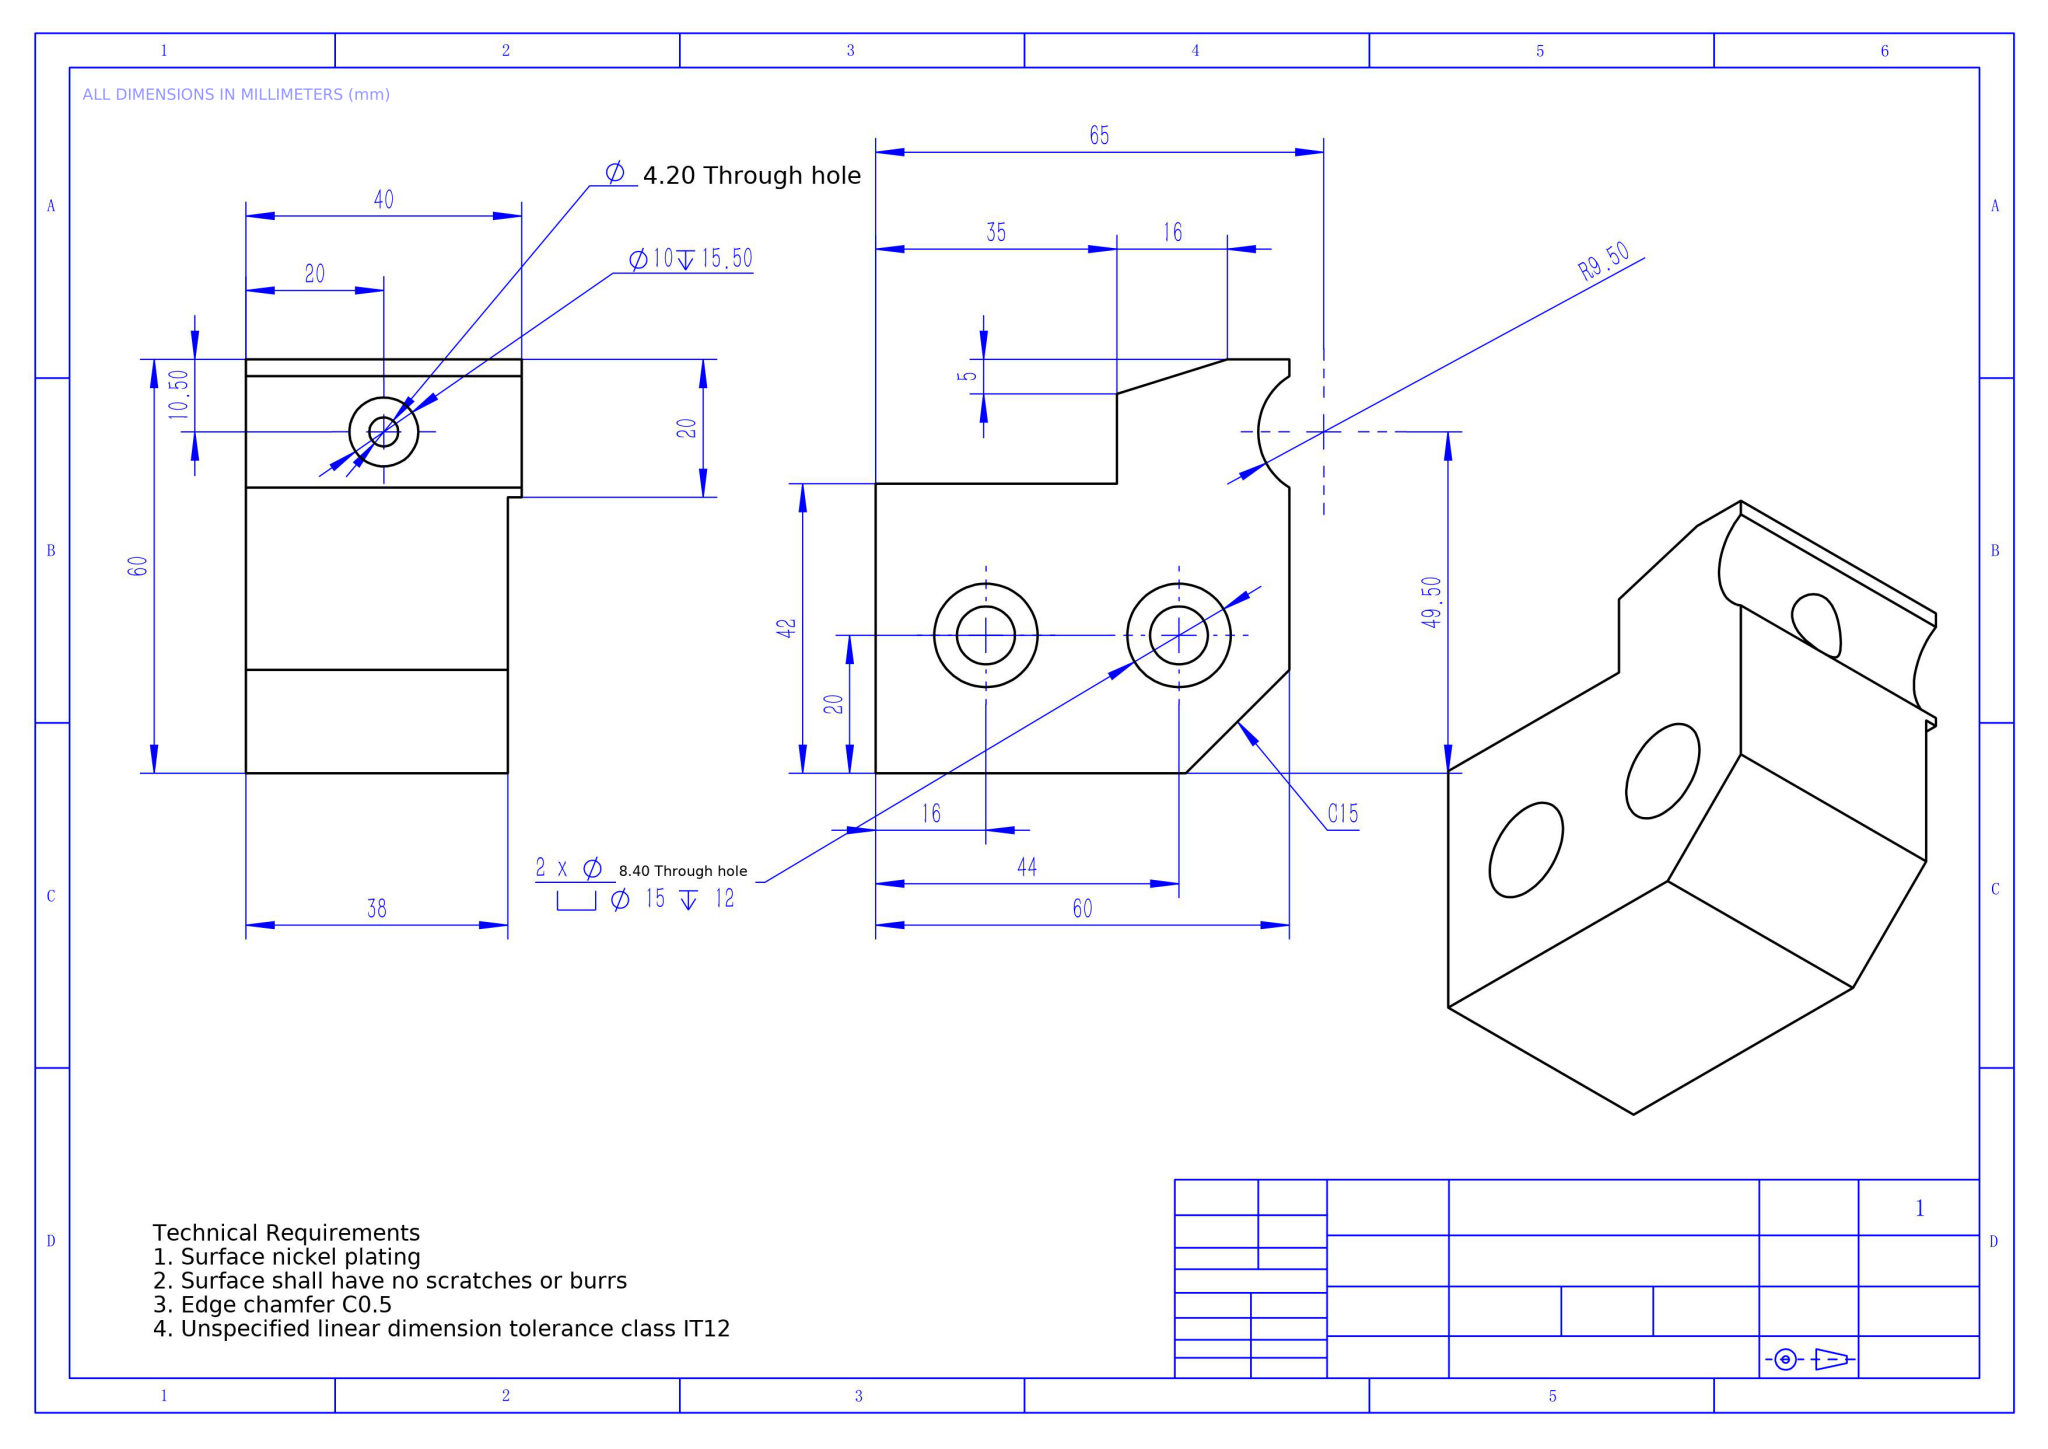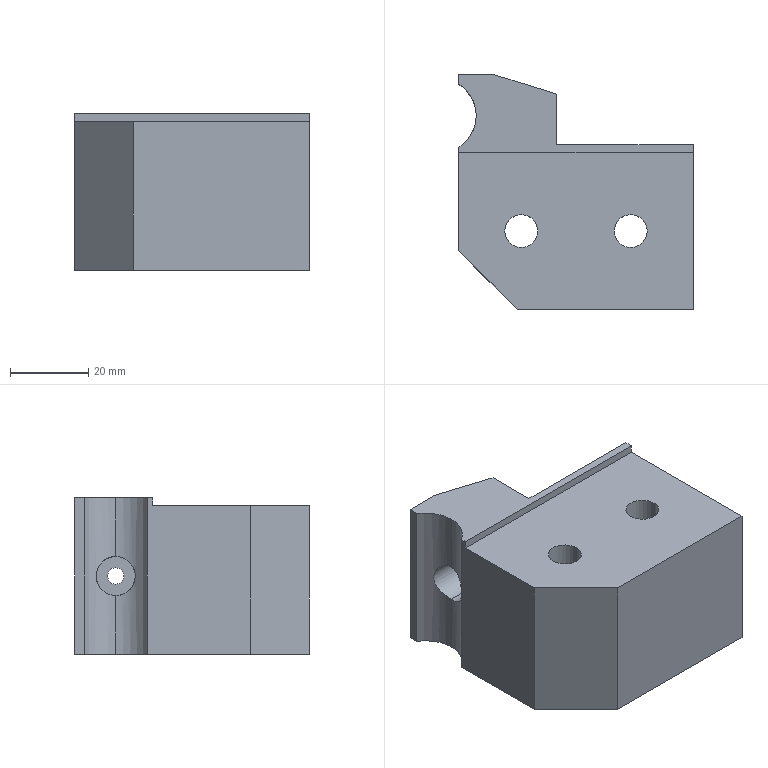Part | NX | mm | 1 solid | 30 faces | box 60 x 60 x 40 mm | volume 97635 mm3 | plane 16 | cylinder 14 | commonest cylinder face diameters 15 x4 8.4 x4 10 x2 19 x2 4.2 x2
STEP:
#1=COLOUR_RGB('',0.698,0.698,0.698);
#2=FILL_AREA_STYLE_COLOUR('',#1);
#3=FILL_AREA_STYLE('',(#2));
#4=SURFACE_STYLE_FILL_AREA(#3);
#5=SURFACE_SIDE_STYLE('',(#4));
#6=SURFACE_STYLE_USAGE(.BOTH.,#5);
#7=PRESENTATION_STYLE_ASSIGNMENT((#6));
#8=CARTESIAN_POINT('',(20.,49.5,15.));
#9=VERTEX_POINT('',#8);
#10=CARTESIAN_POINT('',(20.,49.5,25.));
#11=VERTEX_POINT('',#10);
#12=CARTESIAN_POINT('',(20.,49.5,20.));
#13=DIRECTION('',(-1.,0.,0.));
#14=DIRECTION('',(0.,0.,1.));
#15=AXIS2_PLACEMENT_3D('',#12,#13,#14);
#16=CIRCLE('',#15,5.);
#17=EDGE_CURVE('',#9,#11,#16,.T.);
#18=ORIENTED_EDGE('',*,*,#17,.F.);
#19=CARTESIAN_POINT('',(4.5,49.5,15.));
#20=VERTEX_POINT('',#19);
#21=CARTESIAN_POINT('',(20.,49.5,15.));
#22=DIRECTION('',(-1.,0.,0.));
#23=VECTOR('',#22,1000.);
#24=LINE('',#21,#23);
#25=EDGE_CURVE('',#9,#20,#24,.T.);
#26=ORIENTED_EDGE('',*,*,#25,.T.);
#27=CARTESIAN_POINT('',(4.5,49.5,25.));
#28=VERTEX_POINT('',#27);
#29=CARTESIAN_POINT('',(4.5,49.5,25.));
#30=CARTESIAN_POINT('',(4.5,49.163,25.));
#31=CARTESIAN_POINT('',(4.482,48.832,24.966));
#32=CARTESIAN_POINT('',(4.414,48.184,24.835));
#33=CARTESIAN_POINT('',(4.363,47.863,24.736));
#34=CARTESIAN_POINT('',(4.237,47.259,24.482));
#35=CARTESIAN_POINT('',(4.162,46.974,24.327));
#36=CARTESIAN_POINT('',(3.996,46.435,23.964));
#37=CARTESIAN_POINT('',(3.906,46.186,23.757));
#38=CARTESIAN_POINT('',(3.725,45.734,23.304));
#39=CARTESIAN_POINT('',(3.632,45.528,23.054));
#40=CARTESIAN_POINT('',(3.457,45.168,22.518));
#41=CARTESIAN_POINT('',(3.376,45.015,22.234));
#42=CARTESIAN_POINT('',(3.237,44.764,21.636));
#43=CARTESIAN_POINT('',(3.178,44.665,21.316));
#44=CARTESIAN_POINT('',(3.099,44.534,20.668));
#45=CARTESIAN_POINT('',(3.078,44.5,20.339));
#46=CARTESIAN_POINT('',(3.078,44.5,19.839));
#47=CARTESIAN_POINT('',(3.083,44.508,19.67));
#48=CARTESIAN_POINT('',(3.103,44.541,19.337));
#49=CARTESIAN_POINT('',(3.118,44.566,19.172));
#50=CARTESIAN_POINT('',(3.158,44.632,18.848));
#51=CARTESIAN_POINT('',(3.182,44.672,18.689));
#52=CARTESIAN_POINT('',(3.238,44.769,18.373));
#53=CARTESIAN_POINT('',(3.271,44.826,18.217));
#54=CARTESIAN_POINT('',(3.376,45.016,17.764));
#55=CARTESIAN_POINT('',(3.458,45.17,17.479));
#56=CARTESIAN_POINT('',(3.633,45.53,16.943));
#57=CARTESIAN_POINT('',(3.726,45.737,16.692));
#58=CARTESIAN_POINT('',(3.908,46.19,16.239));
#59=CARTESIAN_POINT('',(3.997,46.438,16.034));
#60=CARTESIAN_POINT('',(4.164,46.979,15.67));
#61=CARTESIAN_POINT('',(4.238,47.264,15.516));
#62=CARTESIAN_POINT('',(4.332,47.714,15.327));
#63=CARTESIAN_POINT('',(4.36,47.868,15.271));
#64=CARTESIAN_POINT('',(4.41,48.184,15.173));
#65=CARTESIAN_POINT('',(4.431,48.347,15.132));
#66=CARTESIAN_POINT('',(4.483,48.837,15.033));
#67=CARTESIAN_POINT('',(4.5,49.167,15.));
#68=CARTESIAN_POINT('',(4.5,49.5,15.));
#69=B_SPLINE_CURVE_WITH_KNOTS('',3,(#29,#30,#31,#32,#33,#34,#35,#36,#37,#38,#39,#40,#41,#42,#43,#44,#45,#46,#47,#48,#49,#50,#51,#52,#53,#54,#55,#56,#57,#58,#59,#60,#61,#62,#63,#64,#65,#66,#67,#68),.UNSPECIFIED.,.F.,.F.,(4,2,2,2,2,2,2,2,2,2,2,2,2,2,2,2,2,2,2,4),(0.,0.0009961,0.001992,0.002988,0.003985,0.004981,0.005977,0.006973,0.007969,0.008467,0.008965,0.009463,0.009961,0.01096,0.01195,0.01295,0.01395,0.01444,0.01494,0.01594),.UNSPECIFIED.);
#70=EDGE_CURVE('',#28,#20,#69,.T.);
#71=ORIENTED_EDGE('',*,*,#70,.F.);
#72=CARTESIAN_POINT('',(20.,49.5,25.));
#73=DIRECTION('',(-1.,0.,0.));
#74=VECTOR('',#73,1000.);
#75=LINE('',#72,#74);
#76=EDGE_CURVE('',#11,#28,#75,.T.);
#77=ORIENTED_EDGE('',*,*,#76,.F.);
#78=EDGE_LOOP('',(#18,#26,#71,#77));
#79=FACE_OUTER_BOUND('',#78,.T.);
#80=CARTESIAN_POINT('',(20.,49.5,20.));
#81=DIRECTION('',(-1.,0.,0.));
#82=DIRECTION('',(0.,0.,1.));
#83=AXIS2_PLACEMENT_3D('',#80,#81,#82);
#84=CYLINDRICAL_SURFACE('',#83,5.);
#85=ADVANCED_FACE('',(#79),#84,.F.);
#86=CARTESIAN_POINT('',(51.5,20.,12.));
#87=VERTEX_POINT('',#86);
#88=CARTESIAN_POINT('',(36.5,20.,12.));
#89=VERTEX_POINT('',#88);
#90=CARTESIAN_POINT('',(44.,20.,12.));
#91=DIRECTION('',(0.,0.,-1.));
#92=DIRECTION('',(-1.,0.,0.));
#93=AXIS2_PLACEMENT_3D('',#90,#91,#92);
#94=CIRCLE('',#93,7.5);
#95=EDGE_CURVE('',#87,#89,#94,.T.);
#96=ORIENTED_EDGE('',*,*,#95,.F.);
#97=CARTESIAN_POINT('',(51.5,20.,0.));
#98=VERTEX_POINT('',#97);
#99=CARTESIAN_POINT('',(51.5,20.,0.));
#100=DIRECTION('',(0.,0.,-1.));
#101=VECTOR('',#100,1000.);
#102=LINE('',#99,#101);
#103=EDGE_CURVE('',#87,#98,#102,.T.);
#104=ORIENTED_EDGE('',*,*,#103,.T.);
#105=CARTESIAN_POINT('',(36.5,20.,0.));
#106=VERTEX_POINT('',#105);
#107=CARTESIAN_POINT('',(44.,20.,0.));
#108=DIRECTION('',(0.,0.,-1.));
#109=DIRECTION('',(-1.,0.,0.));
#110=AXIS2_PLACEMENT_3D('',#107,#108,#109);
#111=CIRCLE('',#110,7.5);
#112=EDGE_CURVE('',#98,#106,#111,.T.);
#113=ORIENTED_EDGE('',*,*,#112,.T.);
#114=CARTESIAN_POINT('',(36.5,20.,0.));
#115=DIRECTION('',(0.,0.,-1.));
#116=VECTOR('',#115,1000.);
#117=LINE('',#114,#116);
#118=EDGE_CURVE('',#89,#106,#117,.T.);
#119=ORIENTED_EDGE('',*,*,#118,.F.);
#120=EDGE_LOOP('',(#96,#104,#113,#119));
#121=FACE_OUTER_BOUND('',#120,.T.);
#122=CARTESIAN_POINT('',(44.,20.,0.));
#123=DIRECTION('',(0.,0.,-1.));
#124=DIRECTION('',(-1.,0.,0.));
#125=AXIS2_PLACEMENT_3D('',#122,#123,#124);
#126=CYLINDRICAL_SURFACE('',#125,7.5);
#127=ADVANCED_FACE('',(#121),#126,.F.);
#128=CARTESIAN_POINT('',(39.8,20.,38.));
#129=VERTEX_POINT('',#128);
#130=CARTESIAN_POINT('',(48.2,20.,38.));
#131=VERTEX_POINT('',#130);
#132=CARTESIAN_POINT('',(44.,20.,38.));
#133=DIRECTION('',(0.,0.,1.));
#134=DIRECTION('',(1.,0.,0.));
#135=AXIS2_PLACEMENT_3D('',#132,#133,#134);
#136=CIRCLE('',#135,4.2);
#137=EDGE_CURVE('',#129,#131,#136,.T.);
#138=ORIENTED_EDGE('',*,*,#137,.T.);
#139=CARTESIAN_POINT('',(48.2,20.,12.));
#140=VERTEX_POINT('',#139);
#141=CARTESIAN_POINT('',(48.2,20.,0.));
#142=DIRECTION('',(0.,0.,-1.));
#143=VECTOR('',#142,1000.);
#144=LINE('',#141,#143);
#145=EDGE_CURVE('',#131,#140,#144,.T.);
#146=ORIENTED_EDGE('',*,*,#145,.T.);
#147=CARTESIAN_POINT('',(39.8,20.,12.));
#148=VERTEX_POINT('',#147);
#149=CARTESIAN_POINT('',(44.,20.,12.));
#150=DIRECTION('',(0.,0.,-1.));
#151=DIRECTION('',(-1.,0.,0.));
#152=AXIS2_PLACEMENT_3D('',#149,#150,#151);
#153=CIRCLE('',#152,4.2);
#154=EDGE_CURVE('',#140,#148,#153,.T.);
#155=ORIENTED_EDGE('',*,*,#154,.T.);
#156=CARTESIAN_POINT('',(39.8,20.,0.));
#157=DIRECTION('',(0.,0.,-1.));
#158=VECTOR('',#157,1000.);
#159=LINE('',#156,#158);
#160=EDGE_CURVE('',#129,#148,#159,.T.);
#161=ORIENTED_EDGE('',*,*,#160,.F.);
#162=EDGE_LOOP('',(#138,#146,#155,#161));
#163=FACE_OUTER_BOUND('',#162,.T.);
#164=CARTESIAN_POINT('',(44.,20.,0.));
#165=DIRECTION('',(0.,0.,-1.));
#166=DIRECTION('',(-1.,0.,0.));
#167=AXIS2_PLACEMENT_3D('',#164,#165,#166);
#168=CYLINDRICAL_SURFACE('',#167,4.2);
#169=ADVANCED_FACE('',(#163),#168,.F.);
#170=CARTESIAN_POINT('',(23.5,20.,12.));
#171=VERTEX_POINT('',#170);
#172=CARTESIAN_POINT('',(8.5,20.,12.));
#173=VERTEX_POINT('',#172);
#174=CARTESIAN_POINT('',(16.,20.,12.));
#175=DIRECTION('',(0.,0.,-1.));
#176=DIRECTION('',(-1.,0.,0.));
#177=AXIS2_PLACEMENT_3D('',#174,#175,#176);
#178=CIRCLE('',#177,7.5);
#179=EDGE_CURVE('',#171,#173,#178,.T.);
#180=ORIENTED_EDGE('',*,*,#179,.F.);
#181=CARTESIAN_POINT('',(23.5,20.,0.));
#182=VERTEX_POINT('',#181);
#183=CARTESIAN_POINT('',(23.5,20.,0.));
#184=DIRECTION('',(0.,0.,-1.));
#185=VECTOR('',#184,1000.);
#186=LINE('',#183,#185);
#187=EDGE_CURVE('',#171,#182,#186,.T.);
#188=ORIENTED_EDGE('',*,*,#187,.T.);
#189=CARTESIAN_POINT('',(8.5,20.,0.));
#190=VERTEX_POINT('',#189);
#191=CARTESIAN_POINT('',(16.,20.,0.));
#192=DIRECTION('',(0.,0.,-1.));
#193=DIRECTION('',(-1.,0.,0.));
#194=AXIS2_PLACEMENT_3D('',#191,#192,#193);
#195=CIRCLE('',#194,7.5);
#196=EDGE_CURVE('',#182,#190,#195,.T.);
#197=ORIENTED_EDGE('',*,*,#196,.T.);
#198=CARTESIAN_POINT('',(8.5,20.,0.));
#199=DIRECTION('',(0.,0.,-1.));
#200=VECTOR('',#199,1000.);
#201=LINE('',#198,#200);
#202=EDGE_CURVE('',#173,#190,#201,.T.);
#203=ORIENTED_EDGE('',*,*,#202,.F.);
#204=EDGE_LOOP('',(#180,#188,#197,#203));
#205=FACE_OUTER_BOUND('',#204,.T.);
#206=CARTESIAN_POINT('',(16.,20.,0.));
#207=DIRECTION('',(0.,0.,-1.));
#208=DIRECTION('',(-1.,0.,0.));
#209=AXIS2_PLACEMENT_3D('',#206,#207,#208);
#210=CYLINDRICAL_SURFACE('',#209,7.5);
#211=ADVANCED_FACE('',(#205),#210,.F.);
#212=CARTESIAN_POINT('',(11.8,20.,38.));
#213=VERTEX_POINT('',#212);
#214=CARTESIAN_POINT('',(20.2,20.,38.));
#215=VERTEX_POINT('',#214);
#216=CARTESIAN_POINT('',(16.,20.,38.));
#217=DIRECTION('',(0.,0.,1.));
#218=DIRECTION('',(1.,0.,0.));
#219=AXIS2_PLACEMENT_3D('',#216,#217,#218);
#220=CIRCLE('',#219,4.2);
#221=EDGE_CURVE('',#213,#215,#220,.T.);
#222=ORIENTED_EDGE('',*,*,#221,.T.);
#223=CARTESIAN_POINT('',(20.2,20.,12.));
#224=VERTEX_POINT('',#223);
#225=CARTESIAN_POINT('',(20.2,20.,0.));
#226=DIRECTION('',(0.,0.,-1.));
#227=VECTOR('',#226,1000.);
#228=LINE('',#225,#227);
#229=EDGE_CURVE('',#215,#224,#228,.T.);
#230=ORIENTED_EDGE('',*,*,#229,.T.);
#231=CARTESIAN_POINT('',(11.8,20.,12.));
#232=VERTEX_POINT('',#231);
#233=CARTESIAN_POINT('',(16.,20.,12.));
#234=DIRECTION('',(0.,0.,-1.));
#235=DIRECTION('',(-1.,0.,0.));
#236=AXIS2_PLACEMENT_3D('',#233,#234,#235);
#237=CIRCLE('',#236,4.2);
#238=EDGE_CURVE('',#224,#232,#237,.T.);
#239=ORIENTED_EDGE('',*,*,#238,.T.);
#240=CARTESIAN_POINT('',(11.8,20.,0.));
#241=DIRECTION('',(0.,0.,-1.));
#242=VECTOR('',#241,1000.);
#243=LINE('',#240,#242);
#244=EDGE_CURVE('',#213,#232,#243,.T.);
#245=ORIENTED_EDGE('',*,*,#244,.F.);
#246=EDGE_LOOP('',(#222,#230,#239,#245));
#247=FACE_OUTER_BOUND('',#246,.T.);
#248=CARTESIAN_POINT('',(16.,20.,0.));
#249=DIRECTION('',(0.,0.,-1.));
#250=DIRECTION('',(-1.,0.,0.));
#251=AXIS2_PLACEMENT_3D('',#248,#249,#250);
#252=CYLINDRICAL_SURFACE('',#251,4.2);
#253=ADVANCED_FACE('',(#247),#252,.F.);
#254=CARTESIAN_POINT('',(0.,57.578,0.));
#255=VERTEX_POINT('',#254);
#256=CARTESIAN_POINT('',(4.5,49.5,0.));
#257=VERTEX_POINT('',#256);
#258=CARTESIAN_POINT('',(-5.,49.5,0.));
#259=DIRECTION('',(0.,0.,-1.));
#260=DIRECTION('',(-1.,0.,0.));
#261=AXIS2_PLACEMENT_3D('',#258,#259,#260);
#262=CIRCLE('',#261,9.5);
#263=EDGE_CURVE('',#255,#257,#262,.T.);
#264=ORIENTED_EDGE('',*,*,#263,.T.);
#265=CARTESIAN_POINT('',(4.5,49.5,0.));
#266=DIRECTION('',(0.,0.,1.));
#267=VECTOR('',#266,1000.);
#268=LINE('',#265,#267);
#269=EDGE_CURVE('',#257,#20,#268,.T.);
#270=ORIENTED_EDGE('',*,*,#269,.T.);
#271=CARTESIAN_POINT('',(4.5,49.5,15.));
#272=CARTESIAN_POINT('',(4.5,49.832,15.));
#273=CARTESIAN_POINT('',(4.482,50.17,15.034));
#274=CARTESIAN_POINT('',(4.414,50.819,15.166));
#275=CARTESIAN_POINT('',(4.363,51.135,15.263));
#276=CARTESIAN_POINT('',(4.237,51.743,15.519));
#277=CARTESIAN_POINT('',(4.162,52.028,15.674));
#278=CARTESIAN_POINT('',(3.997,52.563,16.035));
#279=CARTESIAN_POINT('',(3.906,52.815,16.243));
#280=CARTESIAN_POINT('',(3.725,53.267,16.697));
#281=CARTESIAN_POINT('',(3.633,53.47,16.943));
#282=CARTESIAN_POINT('',(3.458,53.83,17.48));
#283=CARTESIAN_POINT('',(3.376,53.985,17.767));
#284=CARTESIAN_POINT('',(3.237,54.236,18.364));
#285=CARTESIAN_POINT('',(3.179,54.333,18.676));
#286=CARTESIAN_POINT('',(3.099,54.466,19.331));
#287=CARTESIAN_POINT('',(3.078,54.5,19.662));
#288=CARTESIAN_POINT('',(3.078,54.5,20.159));
#289=CARTESIAN_POINT('',(3.083,54.492,20.325));
#290=CARTESIAN_POINT('',(3.103,54.459,20.658));
#291=CARTESIAN_POINT('',(3.118,54.434,20.824));
#292=CARTESIAN_POINT('',(3.177,54.336,21.312));
#293=CARTESIAN_POINT('',(3.234,54.24,21.626));
#294=CARTESIAN_POINT('',(3.375,53.986,22.232));
#295=CARTESIAN_POINT('',(3.457,53.832,22.518));
#296=CARTESIAN_POINT('',(3.632,53.473,23.052));
#297=CARTESIAN_POINT('',(3.725,53.267,23.304));
#298=CARTESIAN_POINT('',(3.907,52.813,23.759));
#299=CARTESIAN_POINT('',(3.996,52.566,23.962));
#300=CARTESIAN_POINT('',(4.161,52.031,24.324));
#301=CARTESIAN_POINT('',(4.237,51.74,24.482));
#302=CARTESIAN_POINT('',(4.362,51.14,24.735));
#303=CARTESIAN_POINT('',(4.413,50.827,24.832));
#304=CARTESIAN_POINT('',(4.482,50.174,24.966));
#305=CARTESIAN_POINT('',(4.5,49.837,25.));
#306=CARTESIAN_POINT('',(4.5,49.5,25.));
#307=B_SPLINE_CURVE_WITH_KNOTS('',3,(#271,#272,#273,#274,#275,#276,#277,#278,#279,#280,#281,#282,#283,#284,#285,#286,#287,#288,#289,#290,#291,#292,#293,#294,#295,#296,#297,#298,#299,#300,#301,#302,#303,#304,#305,#306),.UNSPECIFIED.,.F.,.F.,(4,2,2,2,2,2,2,2,2,2,2,2,2,2,2,2,2,4),(0.01594,0.01693,0.01793,0.01892,0.01991,0.02091,0.0219,0.0229,0.02389,0.02439,0.02488,0.02588,0.02687,0.02787,0.02886,0.02986,0.03085,0.03184),.UNSPECIFIED.);
#308=EDGE_CURVE('',#20,#28,#307,.T.);
#309=ORIENTED_EDGE('',*,*,#308,.T.);
#310=CARTESIAN_POINT('',(4.5,49.5,40.));
#311=VERTEX_POINT('',#310);
#312=CARTESIAN_POINT('',(4.5,49.5,0.));
#313=DIRECTION('',(0.,0.,1.));
#314=VECTOR('',#313,1000.);
#315=LINE('',#312,#314);
#316=EDGE_CURVE('',#28,#311,#315,.T.);
#317=ORIENTED_EDGE('',*,*,#316,.T.);
#318=CARTESIAN_POINT('',(-0.,57.578,40.));
#319=VERTEX_POINT('',#318);
#320=CARTESIAN_POINT('',(-5.,49.5,40.));
#321=DIRECTION('',(0.,0.,1.));
#322=DIRECTION('',(1.,0.,0.));
#323=AXIS2_PLACEMENT_3D('',#320,#321,#322);
#324=CIRCLE('',#323,9.5);
#325=EDGE_CURVE('',#311,#319,#324,.T.);
#326=ORIENTED_EDGE('',*,*,#325,.T.);
#327=CARTESIAN_POINT('',(0.,57.578,0.));
#328=DIRECTION('',(0.,0.,1.));
#329=VECTOR('',#328,1000.);
#330=LINE('',#327,#329);
#331=EDGE_CURVE('',#255,#319,#330,.T.);
#332=ORIENTED_EDGE('',*,*,#331,.F.);
#333=EDGE_LOOP('',(#264,#270,#309,#317,#326,#332));
#334=FACE_OUTER_BOUND('',#333,.T.);
#335=CARTESIAN_POINT('',(-5.,49.5,0.));
#336=DIRECTION('',(0.,0.,1.));
#337=DIRECTION('',(1.,0.,0.));
#338=AXIS2_PLACEMENT_3D('',#335,#336,#337);
#339=CYLINDRICAL_SURFACE('',#338,9.5);
#340=ADVANCED_FACE('',(#334),#339,.F.);
#341=CARTESIAN_POINT('',(20.,49.5,22.1));
#342=VERTEX_POINT('',#341);
#343=CARTESIAN_POINT('',(20.,49.5,17.9));
#344=VERTEX_POINT('',#343);
#345=CARTESIAN_POINT('',(20.,49.5,20.));
#346=DIRECTION('',(1.,0.,0.));
#347=DIRECTION('',(0.,0.,1.));
#348=AXIS2_PLACEMENT_3D('',#345,#346,#347);
#349=CIRCLE('',#348,2.1);
#350=EDGE_CURVE('',#342,#344,#349,.T.);
#351=ORIENTED_EDGE('',*,*,#350,.F.);
#352=CARTESIAN_POINT('',(25.,49.5,22.1));
#353=VERTEX_POINT('',#352);
#354=CARTESIAN_POINT('',(25.,49.5,22.1));
#355=DIRECTION('',(1.,0.,0.));
#356=VECTOR('',#355,1000.);
#357=LINE('',#354,#356);
#358=EDGE_CURVE('',#342,#353,#357,.T.);
#359=ORIENTED_EDGE('',*,*,#358,.T.);
#360=CARTESIAN_POINT('',(25.,49.5,17.9));
#361=VERTEX_POINT('',#360);
#362=CARTESIAN_POINT('',(25.,49.5,20.));
#363=DIRECTION('',(1.,0.,0.));
#364=DIRECTION('',(0.,0.,-1.));
#365=AXIS2_PLACEMENT_3D('',#362,#363,#364);
#366=CIRCLE('',#365,2.1);
#367=EDGE_CURVE('',#353,#361,#366,.T.);
#368=ORIENTED_EDGE('',*,*,#367,.T.);
#369=CARTESIAN_POINT('',(25.,49.5,17.9));
#370=DIRECTION('',(1.,0.,0.));
#371=VECTOR('',#370,1000.);
#372=LINE('',#369,#371);
#373=EDGE_CURVE('',#344,#361,#372,.T.);
#374=ORIENTED_EDGE('',*,*,#373,.F.);
#375=EDGE_LOOP('',(#351,#359,#368,#374));
#376=FACE_OUTER_BOUND('',#375,.T.);
#377=CARTESIAN_POINT('',(25.,49.5,20.));
#378=DIRECTION('',(1.,0.,0.));
#379=DIRECTION('',(0.,0.,-1.));
#380=AXIS2_PLACEMENT_3D('',#377,#378,#379);
#381=CYLINDRICAL_SURFACE('',#380,2.1);
#382=ADVANCED_FACE('',(#376),#381,.F.);
#383=ORIENTED_EDGE('',*,*,#358,.F.);
#384=CARTESIAN_POINT('',(20.,49.5,20.));
#385=DIRECTION('',(1.,0.,0.));
#386=DIRECTION('',(0.,0.,1.));
#387=AXIS2_PLACEMENT_3D('',#384,#385,#386);
#388=CIRCLE('',#387,2.1);
#389=EDGE_CURVE('',#344,#342,#388,.T.);
#390=ORIENTED_EDGE('',*,*,#389,.F.);
#391=ORIENTED_EDGE('',*,*,#373,.T.);
#392=CARTESIAN_POINT('',(25.,49.5,20.));
#393=DIRECTION('',(1.,0.,0.));
#394=DIRECTION('',(0.,0.,-1.));
#395=AXIS2_PLACEMENT_3D('',#392,#393,#394);
#396=CIRCLE('',#395,2.1);
#397=EDGE_CURVE('',#361,#353,#396,.T.);
#398=ORIENTED_EDGE('',*,*,#397,.T.);
#399=EDGE_LOOP('',(#383,#390,#391,#398));
#400=FACE_OUTER_BOUND('',#399,.T.);
#401=CARTESIAN_POINT('',(25.,49.5,20.));
#402=DIRECTION('',(1.,0.,0.));
#403=DIRECTION('',(0.,0.,-1.));
#404=AXIS2_PLACEMENT_3D('',#401,#402,#403);
#405=CYLINDRICAL_SURFACE('',#404,2.1);
#406=ADVANCED_FACE('',(#400),#405,.F.);
#407=CARTESIAN_POINT('',(15.,-0.,38.));
#408=VERTEX_POINT('',#407);
#409=CARTESIAN_POINT('',(60.,0.,38.));
#410=VERTEX_POINT('',#409);
#411=CARTESIAN_POINT('',(60.,0.,38.));
#412=DIRECTION('',(1.,0.,0.));
#413=VECTOR('',#412,1000.);
#414=LINE('',#411,#413);
#415=EDGE_CURVE('',#408,#410,#414,.T.);
#416=ORIENTED_EDGE('',*,*,#415,.F.);
#417=CARTESIAN_POINT('',(15.,0.,0.));
#418=VERTEX_POINT('',#417);
#419=CARTESIAN_POINT('',(15.,0.,40.));
#420=DIRECTION('',(0.,0.,-1.));
#421=VECTOR('',#420,1000.);
#422=LINE('',#419,#421);
#423=EDGE_CURVE('',#408,#418,#422,.T.);
#424=ORIENTED_EDGE('',*,*,#423,.T.);
#425=CARTESIAN_POINT('',(60.,0.,0.));
#426=VERTEX_POINT('',#425);
#427=CARTESIAN_POINT('',(0.,0.,0.));
#428=DIRECTION('',(1.,0.,0.));
#429=VECTOR('',#428,1000.);
#430=LINE('',#427,#429);
#431=EDGE_CURVE('',#418,#426,#430,.T.);
#432=ORIENTED_EDGE('',*,*,#431,.T.);
#433=CARTESIAN_POINT('',(60.,0.,40.));
#434=DIRECTION('',(0.,0.,-1.));
#435=VECTOR('',#434,1000.);
#436=LINE('',#433,#435);
#437=EDGE_CURVE('',#410,#426,#436,.T.);
#438=ORIENTED_EDGE('',*,*,#437,.F.);
#439=EDGE_LOOP('',(#416,#424,#432,#438));
#440=FACE_OUTER_BOUND('',#439,.T.);
#441=CARTESIAN_POINT('',(0.,0.,40.));
#442=DIRECTION('',(0.,1.,0.));
#443=DIRECTION('',(0.,0.,1.));
#444=AXIS2_PLACEMENT_3D('',#441,#442,#443);
#445=PLANE('',#444);
#446=ADVANCED_FACE('',(#440),#445,.F.);
#447=ORIENTED_EDGE('',*,*,#423,.F.);
#448=CARTESIAN_POINT('',(0.,15.,38.));
#449=VERTEX_POINT('',#448);
#450=CARTESIAN_POINT('',(15.,0.,38.));
#451=DIRECTION('',(-0.7071,0.7071,0.));
#452=VECTOR('',#451,1000.);
#453=LINE('',#450,#452);
#454=EDGE_CURVE('',#408,#449,#453,.T.);
#455=ORIENTED_EDGE('',*,*,#454,.T.);
#456=CARTESIAN_POINT('',(0.,15.,0.));
#457=VERTEX_POINT('',#456);
#458=CARTESIAN_POINT('',(0.,15.,40.));
#459=DIRECTION('',(0.,0.,1.));
#460=VECTOR('',#459,1000.);
#461=LINE('',#458,#460);
#462=EDGE_CURVE('',#457,#449,#461,.T.);
#463=ORIENTED_EDGE('',*,*,#462,.F.);
#464=CARTESIAN_POINT('',(7.5,7.5,0.));
#465=DIRECTION('',(-0.7071,0.7071,0.));
#466=VECTOR('',#465,1000.);
#467=LINE('',#464,#466);
#468=EDGE_CURVE('',#418,#457,#467,.T.);
#469=ORIENTED_EDGE('',*,*,#468,.F.);
#470=EDGE_LOOP('',(#447,#455,#463,#469));
#471=FACE_OUTER_BOUND('',#470,.T.);
#472=CARTESIAN_POINT('',(15.,0.,40.));
#473=DIRECTION('',(0.7071,0.7071,0.));
#474=DIRECTION('',(0.,0.,-1.));
#475=AXIS2_PLACEMENT_3D('',#472,#473,#474);
#476=PLANE('',#475);
#477=ADVANCED_FACE('',(#471),#476,.F.);
#478=CARTESIAN_POINT('',(0.,60.,0.));
#479=VERTEX_POINT('',#478);
#480=CARTESIAN_POINT('',(0.,0.,0.));
#481=DIRECTION('',(0.,-1.,0.));
#482=VECTOR('',#481,1000.);
#483=LINE('',#480,#482);
#484=EDGE_CURVE('',#479,#255,#483,.T.);
#485=ORIENTED_EDGE('',*,*,#484,.T.);
#486=ORIENTED_EDGE('',*,*,#331,.T.);
#487=CARTESIAN_POINT('',(0.,60.,40.));
#488=VERTEX_POINT('',#487);
#489=CARTESIAN_POINT('',(0.,0.,40.));
#490=DIRECTION('',(0.,-1.,0.));
#491=VECTOR('',#490,1000.);
#492=LINE('',#489,#491);
#493=EDGE_CURVE('',#488,#319,#492,.T.);
#494=ORIENTED_EDGE('',*,*,#493,.F.);
#495=CARTESIAN_POINT('',(0.,60.,40.));
#496=DIRECTION('',(0.,0.,-1.));
#497=VECTOR('',#496,1000.);
#498=LINE('',#495,#497);
#499=EDGE_CURVE('',#488,#479,#498,.T.);
#500=ORIENTED_EDGE('',*,*,#499,.T.);
#501=EDGE_LOOP('',(#485,#486,#494,#500));
#502=FACE_OUTER_BOUND('',#501,.T.);
#503=CARTESIAN_POINT('',(0.,0.,40.));
#504=DIRECTION('',(1.,0.,0.));
#505=DIRECTION('',(0.,0.,-1.));
#506=AXIS2_PLACEMENT_3D('',#503,#504,#505);
#507=PLANE('',#506);
#508=ADVANCED_FACE('',(#502),#507,.F.);
#509=CARTESIAN_POINT('',(0.,40.,38.));
#510=VERTEX_POINT('',#509);
#511=CARTESIAN_POINT('',(0.,0.,38.));
#512=DIRECTION('',(0.,-1.,0.));
#513=VECTOR('',#512,1000.);
#514=LINE('',#511,#513);
#515=EDGE_CURVE('',#510,#449,#514,.T.);
#516=ORIENTED_EDGE('',*,*,#515,.F.);
#517=CARTESIAN_POINT('',(0.,40.,40.));
#518=VERTEX_POINT('',#517);
#519=CARTESIAN_POINT('',(0.,40.,40.));
#520=DIRECTION('',(0.,0.,1.));
#521=VECTOR('',#520,1000.);
#522=LINE('',#519,#521);
#523=EDGE_CURVE('',#510,#518,#522,.T.);
#524=ORIENTED_EDGE('',*,*,#523,.T.);
#525=CARTESIAN_POINT('',(-0.,41.422,40.));
#526=VERTEX_POINT('',#525);
#527=CARTESIAN_POINT('',(0.,0.,40.));
#528=DIRECTION('',(0.,-1.,0.));
#529=VECTOR('',#528,1000.);
#530=LINE('',#527,#529);
#531=EDGE_CURVE('',#526,#518,#530,.T.);
#532=ORIENTED_EDGE('',*,*,#531,.F.);
#533=CARTESIAN_POINT('',(-0.,41.422,0.));
#534=VERTEX_POINT('',#533);
#535=CARTESIAN_POINT('',(0.,41.422,0.));
#536=DIRECTION('',(0.,0.,-1.));
#537=VECTOR('',#536,1000.);
#538=LINE('',#535,#537);
#539=EDGE_CURVE('',#526,#534,#538,.T.);
#540=ORIENTED_EDGE('',*,*,#539,.T.);
#541=CARTESIAN_POINT('',(0.,0.,0.));
#542=DIRECTION('',(0.,-1.,0.));
#543=VECTOR('',#542,1000.);
#544=LINE('',#541,#543);
#545=EDGE_CURVE('',#534,#457,#544,.T.);
#546=ORIENTED_EDGE('',*,*,#545,.T.);
#547=ORIENTED_EDGE('',*,*,#462,.T.);
#548=EDGE_LOOP('',(#516,#524,#532,#540,#546,#547));
#549=FACE_OUTER_BOUND('',#548,.T.);
#550=CARTESIAN_POINT('',(0.,0.,40.));
#551=DIRECTION('',(1.,0.,0.));
#552=DIRECTION('',(0.,0.,-1.));
#553=AXIS2_PLACEMENT_3D('',#550,#551,#552);
#554=PLANE('',#553);
#555=ADVANCED_FACE('',(#549),#554,.F.);
#556=CARTESIAN_POINT('',(60.,40.,40.));
#557=VERTEX_POINT('',#556);
#558=CARTESIAN_POINT('',(60.,42.,40.));
#559=VERTEX_POINT('',#558);
#560=CARTESIAN_POINT('',(60.,0.,40.));
#561=DIRECTION('',(0.,1.,0.));
#562=VECTOR('',#561,1000.);
#563=LINE('',#560,#562);
#564=EDGE_CURVE('',#557,#559,#563,.T.);
#565=ORIENTED_EDGE('',*,*,#564,.F.);
#566=CARTESIAN_POINT('',(60.,40.,38.));
#567=VERTEX_POINT('',#566);
#568=CARTESIAN_POINT('',(60.,40.,38.));
#569=DIRECTION('',(0.,0.,1.));
#570=VECTOR('',#569,1000.);
#571=LINE('',#568,#570);
#572=EDGE_CURVE('',#567,#557,#571,.T.);
#573=ORIENTED_EDGE('',*,*,#572,.F.);
#574=CARTESIAN_POINT('',(60.,0.,38.));
#575=DIRECTION('',(0.,1.,0.));
#576=VECTOR('',#575,1000.);
#577=LINE('',#574,#576);
#578=EDGE_CURVE('',#410,#567,#577,.T.);
#579=ORIENTED_EDGE('',*,*,#578,.F.);
#580=ORIENTED_EDGE('',*,*,#437,.T.);
#581=CARTESIAN_POINT('',(60.,42.,0.));
#582=VERTEX_POINT('',#581);
#583=CARTESIAN_POINT('',(60.,0.,0.));
#584=DIRECTION('',(0.,1.,0.));
#585=VECTOR('',#584,1000.);
#586=LINE('',#583,#585);
#587=EDGE_CURVE('',#426,#582,#586,.T.);
#588=ORIENTED_EDGE('',*,*,#587,.T.);
#589=CARTESIAN_POINT('',(60.,42.,0.));
#590=DIRECTION('',(0.,0.,1.));
#591=VECTOR('',#590,1000.);
#592=LINE('',#589,#591);
#593=EDGE_CURVE('',#582,#559,#592,.T.);
#594=ORIENTED_EDGE('',*,*,#593,.T.);
#595=EDGE_LOOP('',(#565,#573,#579,#580,#588,#594));
#596=FACE_OUTER_BOUND('',#595,.T.);
#597=CARTESIAN_POINT('',(60.,0.,40.));
#598=DIRECTION('',(-1.,0.,0.));
#599=DIRECTION('',(0.,0.,1.));
#600=AXIS2_PLACEMENT_3D('',#597,#598,#599);
#601=PLANE('',#600);
#602=ADVANCED_FACE('',(#596),#601,.F.);
#603=CARTESIAN_POINT('',(9.,60.,40.));
#604=VERTEX_POINT('',#603);
#605=CARTESIAN_POINT('',(0.,60.,40.));
#606=DIRECTION('',(-1.,0.,0.));
#607=VECTOR('',#606,1000.);
#608=LINE('',#605,#607);
#609=EDGE_CURVE('',#604,#488,#608,.T.);
#610=ORIENTED_EDGE('',*,*,#609,.F.);
#611=CARTESIAN_POINT('',(9.,60.,0.));
#612=VERTEX_POINT('',#611);
#613=CARTESIAN_POINT('',(9.,60.,0.));
#614=DIRECTION('',(0.,0.,1.));
#615=VECTOR('',#614,1000.);
#616=LINE('',#613,#615);
#617=EDGE_CURVE('',#612,#604,#616,.T.);
#618=ORIENTED_EDGE('',*,*,#617,.F.);
#619=CARTESIAN_POINT('',(0.,60.,0.));
#620=DIRECTION('',(-1.,0.,0.));
#621=VECTOR('',#620,1000.);
#622=LINE('',#619,#621);
#623=EDGE_CURVE('',#612,#479,#622,.T.);
#624=ORIENTED_EDGE('',*,*,#623,.T.);
#625=ORIENTED_EDGE('',*,*,#499,.F.);
#626=EDGE_LOOP('',(#610,#618,#624,#625));
#627=FACE_OUTER_BOUND('',#626,.T.);
#628=CARTESIAN_POINT('',(0.,60.,40.));
#629=DIRECTION('',(0.,-1.,0.));
#630=DIRECTION('',(0.,0.,-1.));
#631=AXIS2_PLACEMENT_3D('',#628,#629,#630);
#632=PLANE('',#631);
#633=ADVANCED_FACE('',(#627),#632,.F.);
#634=ORIENTED_EDGE('',*,*,#531,.T.);
#635=CARTESIAN_POINT('',(60.,40.,40.));
#636=DIRECTION('',(-1.,-0.,0.));
#637=VECTOR('',#636,1000.);
#638=LINE('',#635,#637);
#639=EDGE_CURVE('',#557,#518,#638,.T.);
#640=ORIENTED_EDGE('',*,*,#639,.F.);
#641=ORIENTED_EDGE('',*,*,#564,.T.);
#642=CARTESIAN_POINT('',(25.,42.,40.));
#643=VERTEX_POINT('',#642);
#644=CARTESIAN_POINT('',(60.,42.,40.));
#645=DIRECTION('',(1.,0.,0.));
#646=VECTOR('',#645,1000.);
#647=LINE('',#644,#646);
#648=EDGE_CURVE('',#643,#559,#647,.T.);
#649=ORIENTED_EDGE('',*,*,#648,.F.);
#650=CARTESIAN_POINT('',(25.,55.,40.));
#651=VERTEX_POINT('',#650);
#652=CARTESIAN_POINT('',(25.,60.,40.));
#653=DIRECTION('',(0.,-1.,0.));
#654=VECTOR('',#653,1000.);
#655=LINE('',#652,#654);
#656=EDGE_CURVE('',#651,#643,#655,.T.);
#657=ORIENTED_EDGE('',*,*,#656,.F.);
#658=CARTESIAN_POINT('',(9.,60.,40.));
#659=DIRECTION('',(0.9545,-0.2983,0.));
#660=VECTOR('',#659,1000.);
#661=LINE('',#658,#660);
#662=EDGE_CURVE('',#604,#651,#661,.T.);
#663=ORIENTED_EDGE('',*,*,#662,.F.);
#664=ORIENTED_EDGE('',*,*,#609,.T.);
#665=ORIENTED_EDGE('',*,*,#493,.T.);
#666=ORIENTED_EDGE('',*,*,#325,.F.);
#667=CARTESIAN_POINT('',(-5.,49.5,40.));
#668=DIRECTION('',(0.,0.,1.));
#669=DIRECTION('',(1.,0.,0.));
#670=AXIS2_PLACEMENT_3D('',#667,#668,#669);
#671=CIRCLE('',#670,9.5);
#672=EDGE_CURVE('',#526,#311,#671,.T.);
#673=ORIENTED_EDGE('',*,*,#672,.F.);
#674=EDGE_LOOP('',(#634,#640,#641,#649,#657,#663,#664,#665,#666,#673));
#675=FACE_OUTER_BOUND('',#674,.T.);
#676=CARTESIAN_POINT('',(0.,0.,40.));
#677=DIRECTION('',(0.,0.,-1.));
#678=DIRECTION('',(-1.,0.,0.));
#679=AXIS2_PLACEMENT_3D('',#676,#677,#678);
#680=PLANE('',#679);
#681=ADVANCED_FACE('',(#675),#680,.F.);
#682=CARTESIAN_POINT('',(44.,20.,0.));
#683=DIRECTION('',(0.,0.,-1.));
#684=DIRECTION('',(-1.,0.,0.));
#685=AXIS2_PLACEMENT_3D('',#682,#683,#684);
#686=CIRCLE('',#685,7.5);
#687=EDGE_CURVE('',#106,#98,#686,.T.);
#688=ORIENTED_EDGE('',*,*,#687,.F.);
#689=ORIENTED_EDGE('',*,*,#112,.F.);
#690=EDGE_LOOP('',(#688,#689));
#691=FACE_BOUND('',#690,.T.);
#692=CARTESIAN_POINT('',(16.,20.,0.));
#693=DIRECTION('',(0.,0.,-1.));
#694=DIRECTION('',(-1.,0.,0.));
#695=AXIS2_PLACEMENT_3D('',#692,#693,#694);
#696=CIRCLE('',#695,7.5);
#697=EDGE_CURVE('',#190,#182,#696,.T.);
#698=ORIENTED_EDGE('',*,*,#697,.F.);
#699=ORIENTED_EDGE('',*,*,#196,.F.);
#700=EDGE_LOOP('',(#698,#699));
#701=FACE_BOUND('',#700,.T.);
#702=ORIENTED_EDGE('',*,*,#431,.F.);
#703=ORIENTED_EDGE('',*,*,#468,.T.);
#704=ORIENTED_EDGE('',*,*,#545,.F.);
#705=CARTESIAN_POINT('',(-5.,49.5,0.));
#706=DIRECTION('',(0.,0.,-1.));
#707=DIRECTION('',(-1.,0.,0.));
#708=AXIS2_PLACEMENT_3D('',#705,#706,#707);
#709=CIRCLE('',#708,9.5);
#710=EDGE_CURVE('',#257,#534,#709,.T.);
#711=ORIENTED_EDGE('',*,*,#710,.F.);
#712=ORIENTED_EDGE('',*,*,#263,.F.);
#713=ORIENTED_EDGE('',*,*,#484,.F.);
#714=ORIENTED_EDGE('',*,*,#623,.F.);
#715=CARTESIAN_POINT('',(25.,55.,0.));
#716=VERTEX_POINT('',#715);
#717=CARTESIAN_POINT('',(9.,60.,0.));
#718=DIRECTION('',(0.9545,-0.2983,0.));
#719=VECTOR('',#718,1000.);
#720=LINE('',#717,#719);
#721=EDGE_CURVE('',#612,#716,#720,.T.);
#722=ORIENTED_EDGE('',*,*,#721,.T.);
#723=CARTESIAN_POINT('',(25.,42.,0.));
#724=VERTEX_POINT('',#723);
#725=CARTESIAN_POINT('',(25.,60.,0.));
#726=DIRECTION('',(0.,-1.,0.));
#727=VECTOR('',#726,1000.);
#728=LINE('',#725,#727);
#729=EDGE_CURVE('',#716,#724,#728,.T.);
#730=ORIENTED_EDGE('',*,*,#729,.T.);
#731=CARTESIAN_POINT('',(60.,42.,0.));
#732=DIRECTION('',(1.,0.,0.));
#733=VECTOR('',#732,1000.);
#734=LINE('',#731,#733);
#735=EDGE_CURVE('',#724,#582,#734,.T.);
#736=ORIENTED_EDGE('',*,*,#735,.T.);
#737=ORIENTED_EDGE('',*,*,#587,.F.);
#738=EDGE_LOOP('',(#702,#703,#704,#711,#712,#713,#714,#722,#730,#736,#737));
#739=FACE_OUTER_BOUND('',#738,.T.);
#740=CARTESIAN_POINT('',(0.,0.,0.));
#741=DIRECTION('',(0.,0.,-1.));
#742=DIRECTION('',(-1.,0.,0.));
#743=AXIS2_PLACEMENT_3D('',#740,#741,#742);
#744=PLANE('',#743);
#745=ADVANCED_FACE('',(#691,#701,#739),#744,.T.);
#746=ORIENTED_EDGE('',*,*,#648,.T.);
#747=ORIENTED_EDGE('',*,*,#593,.F.);
#748=ORIENTED_EDGE('',*,*,#735,.F.);
#749=CARTESIAN_POINT('',(25.,42.,0.));
#750=DIRECTION('',(0.,0.,1.));
#751=VECTOR('',#750,1000.);
#752=LINE('',#749,#751);
#753=EDGE_CURVE('',#724,#643,#752,.T.);
#754=ORIENTED_EDGE('',*,*,#753,.T.);
#755=EDGE_LOOP('',(#746,#747,#748,#754));
#756=FACE_OUTER_BOUND('',#755,.T.);
#757=CARTESIAN_POINT('',(60.,42.,0.));
#758=DIRECTION('',(0.,-1.,0.));
#759=DIRECTION('',(1.,0.,0.));
#760=AXIS2_PLACEMENT_3D('',#757,#758,#759);
#761=PLANE('',#760);
#762=ADVANCED_FACE('',(#756),#761,.F.);
#763=ORIENTED_EDGE('',*,*,#397,.F.);
#764=ORIENTED_EDGE('',*,*,#367,.F.);
#765=EDGE_LOOP('',(#763,#764));
#766=FACE_BOUND('',#765,.T.);
#767=ORIENTED_EDGE('',*,*,#729,.F.);
#768=CARTESIAN_POINT('',(25.,55.,0.));
#769=DIRECTION('',(0.,0.,1.));
#770=VECTOR('',#769,1000.);
#771=LINE('',#768,#770);
#772=EDGE_CURVE('',#716,#651,#771,.T.);
#773=ORIENTED_EDGE('',*,*,#772,.T.);
#774=ORIENTED_EDGE('',*,*,#656,.T.);
#775=ORIENTED_EDGE('',*,*,#753,.F.);
#776=EDGE_LOOP('',(#767,#773,#774,#775));
#777=FACE_OUTER_BOUND('',#776,.T.);
#778=CARTESIAN_POINT('',(25.,60.,0.));
#779=DIRECTION('',(-1.,0.,0.));
#780=DIRECTION('',(0.,0.,1.));
#781=AXIS2_PLACEMENT_3D('',#778,#779,#780);
#782=PLANE('',#781);
#783=ADVANCED_FACE('',(#766,#777),#782,.F.);
#784=ORIENTED_EDGE('',*,*,#269,.F.);
#785=ORIENTED_EDGE('',*,*,#710,.T.);
#786=ORIENTED_EDGE('',*,*,#539,.F.);
#787=ORIENTED_EDGE('',*,*,#672,.T.);
#788=ORIENTED_EDGE('',*,*,#316,.F.);
#789=ORIENTED_EDGE('',*,*,#70,.T.);
#790=EDGE_LOOP('',(#784,#785,#786,#787,#788,#789));
#791=FACE_OUTER_BOUND('',#790,.T.);
#792=CARTESIAN_POINT('',(-5.,49.5,0.));
#793=DIRECTION('',(0.,0.,1.));
#794=DIRECTION('',(1.,0.,0.));
#795=AXIS2_PLACEMENT_3D('',#792,#793,#794);
#796=CYLINDRICAL_SURFACE('',#795,9.5);
#797=ADVANCED_FACE('',(#791),#796,.F.);
#798=ORIENTED_EDGE('',*,*,#662,.T.);
#799=ORIENTED_EDGE('',*,*,#772,.F.);
#800=ORIENTED_EDGE('',*,*,#721,.F.);
#801=ORIENTED_EDGE('',*,*,#617,.T.);
#802=EDGE_LOOP('',(#798,#799,#800,#801));
#803=FACE_OUTER_BOUND('',#802,.T.);
#804=CARTESIAN_POINT('',(9.,60.,0.));
#805=DIRECTION('',(-0.2983,-0.9545,0.));
#806=DIRECTION('',(0.9545,-0.2983,0.));
#807=AXIS2_PLACEMENT_3D('',#804,#805,#806);
#808=PLANE('',#807);
#809=ADVANCED_FACE('',(#803),#808,.F.);
#810=CARTESIAN_POINT('',(60.,40.,38.));
#811=DIRECTION('',(-1.,-0.,0.));
#812=VECTOR('',#811,1000.);
#813=LINE('',#810,#812);
#814=EDGE_CURVE('',#567,#510,#813,.T.);
#815=ORIENTED_EDGE('',*,*,#814,.F.);
#816=ORIENTED_EDGE('',*,*,#572,.T.);
#817=ORIENTED_EDGE('',*,*,#639,.T.);
#818=ORIENTED_EDGE('',*,*,#523,.F.);
#819=EDGE_LOOP('',(#815,#816,#817,#818));
#820=FACE_OUTER_BOUND('',#819,.T.);
#821=CARTESIAN_POINT('',(60.,40.,38.));
#822=DIRECTION('',(-0.,1.,0.));
#823=DIRECTION('',(-1.,-0.,0.));
#824=AXIS2_PLACEMENT_3D('',#821,#822,#823);
#825=PLANE('',#824);
#826=ADVANCED_FACE('',(#820),#825,.F.);
#827=ORIENTED_EDGE('',*,*,#137,.F.);
#828=CARTESIAN_POINT('',(44.,20.,38.));
#829=DIRECTION('',(0.,0.,1.));
#830=DIRECTION('',(1.,0.,0.));
#831=AXIS2_PLACEMENT_3D('',#828,#829,#830);
#832=CIRCLE('',#831,4.2);
#833=EDGE_CURVE('',#131,#129,#832,.T.);
#834=ORIENTED_EDGE('',*,*,#833,.F.);
#835=EDGE_LOOP('',(#827,#834));
#836=FACE_BOUND('',#835,.T.);
#837=ORIENTED_EDGE('',*,*,#221,.F.);
#838=CARTESIAN_POINT('',(16.,20.,38.));
#839=DIRECTION('',(0.,0.,1.));
#840=DIRECTION('',(1.,0.,0.));
#841=AXIS2_PLACEMENT_3D('',#838,#839,#840);
#842=CIRCLE('',#841,4.2);
#843=EDGE_CURVE('',#215,#213,#842,.T.);
#844=ORIENTED_EDGE('',*,*,#843,.F.);
#845=EDGE_LOOP('',(#837,#844));
#846=FACE_BOUND('',#845,.T.);
#847=ORIENTED_EDGE('',*,*,#515,.T.);
#848=ORIENTED_EDGE('',*,*,#454,.F.);
#849=ORIENTED_EDGE('',*,*,#415,.T.);
#850=ORIENTED_EDGE('',*,*,#578,.T.);
#851=ORIENTED_EDGE('',*,*,#814,.T.);
#852=EDGE_LOOP('',(#847,#848,#849,#850,#851));
#853=FACE_OUTER_BOUND('',#852,.T.);
#854=CARTESIAN_POINT('',(0.,0.,38.));
#855=DIRECTION('',(0.,0.,1.));
#856=DIRECTION('',(1.,0.,0.));
#857=AXIS2_PLACEMENT_3D('',#854,#855,#856);
#858=PLANE('',#857);
#859=ADVANCED_FACE('',(#836,#846,#853),#858,.T.);
#860=ORIENTED_EDGE('',*,*,#229,.F.);
#861=ORIENTED_EDGE('',*,*,#843,.T.);
#862=ORIENTED_EDGE('',*,*,#244,.T.);
#863=CARTESIAN_POINT('',(16.,20.,12.));
#864=DIRECTION('',(0.,0.,-1.));
#865=DIRECTION('',(-1.,0.,0.));
#866=AXIS2_PLACEMENT_3D('',#863,#864,#865);
#867=CIRCLE('',#866,4.2);
#868=EDGE_CURVE('',#232,#224,#867,.T.);
#869=ORIENTED_EDGE('',*,*,#868,.T.);
#870=EDGE_LOOP('',(#860,#861,#862,#869));
#871=FACE_OUTER_BOUND('',#870,.T.);
#872=CARTESIAN_POINT('',(16.,20.,0.));
#873=DIRECTION('',(0.,0.,-1.));
#874=DIRECTION('',(-1.,0.,0.));
#875=AXIS2_PLACEMENT_3D('',#872,#873,#874);
#876=CYLINDRICAL_SURFACE('',#875,4.2);
#877=ADVANCED_FACE('',(#871),#876,.F.);
#878=ORIENTED_EDGE('',*,*,#868,.F.);
#879=ORIENTED_EDGE('',*,*,#238,.F.);
#880=EDGE_LOOP('',(#878,#879));
#881=FACE_BOUND('',#880,.T.);
#882=CARTESIAN_POINT('',(16.,20.,12.));
#883=DIRECTION('',(0.,0.,-1.));
#884=DIRECTION('',(-1.,0.,0.));
#885=AXIS2_PLACEMENT_3D('',#882,#883,#884);
#886=CIRCLE('',#885,7.5);
#887=EDGE_CURVE('',#173,#171,#886,.T.);
#888=ORIENTED_EDGE('',*,*,#887,.T.);
#889=ORIENTED_EDGE('',*,*,#179,.T.);
#890=EDGE_LOOP('',(#888,#889));
#891=FACE_OUTER_BOUND('',#890,.T.);
#892=CARTESIAN_POINT('',(20.2,20.,12.));
#893=DIRECTION('',(0.,0.,1.));
#894=DIRECTION('',(1.,0.,0.));
#895=AXIS2_PLACEMENT_3D('',#892,#893,#894);
#896=PLANE('',#895);
#897=ADVANCED_FACE('',(#881,#891),#896,.F.);
#898=ORIENTED_EDGE('',*,*,#187,.F.);
#899=ORIENTED_EDGE('',*,*,#887,.F.);
#900=ORIENTED_EDGE('',*,*,#202,.T.);
#901=ORIENTED_EDGE('',*,*,#697,.T.);
#902=EDGE_LOOP('',(#898,#899,#900,#901));
#903=FACE_OUTER_BOUND('',#902,.T.);
#904=CARTESIAN_POINT('',(16.,20.,0.));
#905=DIRECTION('',(0.,0.,-1.));
#906=DIRECTION('',(-1.,0.,0.));
#907=AXIS2_PLACEMENT_3D('',#904,#905,#906);
#908=CYLINDRICAL_SURFACE('',#907,7.5);
#909=ADVANCED_FACE('',(#903),#908,.F.);
#910=ORIENTED_EDGE('',*,*,#145,.F.);
#911=ORIENTED_EDGE('',*,*,#833,.T.);
#912=ORIENTED_EDGE('',*,*,#160,.T.);
#913=CARTESIAN_POINT('',(44.,20.,12.));
#914=DIRECTION('',(0.,0.,-1.));
#915=DIRECTION('',(-1.,0.,0.));
#916=AXIS2_PLACEMENT_3D('',#913,#914,#915);
#917=CIRCLE('',#916,4.2);
#918=EDGE_CURVE('',#148,#140,#917,.T.);
#919=ORIENTED_EDGE('',*,*,#918,.T.);
#920=EDGE_LOOP('',(#910,#911,#912,#919));
#921=FACE_OUTER_BOUND('',#920,.T.);
#922=CARTESIAN_POINT('',(44.,20.,0.));
#923=DIRECTION('',(0.,0.,-1.));
#924=DIRECTION('',(-1.,0.,0.));
#925=AXIS2_PLACEMENT_3D('',#922,#923,#924);
#926=CYLINDRICAL_SURFACE('',#925,4.2);
#927=ADVANCED_FACE('',(#921),#926,.F.);
#928=ORIENTED_EDGE('',*,*,#918,.F.);
#929=ORIENTED_EDGE('',*,*,#154,.F.);
#930=EDGE_LOOP('',(#928,#929));
#931=FACE_BOUND('',#930,.T.);
#932=CARTESIAN_POINT('',(44.,20.,12.));
#933=DIRECTION('',(0.,0.,-1.));
#934=DIRECTION('',(-1.,0.,0.));
#935=AXIS2_PLACEMENT_3D('',#932,#933,#934);
#936=CIRCLE('',#935,7.5);
#937=EDGE_CURVE('',#89,#87,#936,.T.);
#938=ORIENTED_EDGE('',*,*,#937,.T.);
#939=ORIENTED_EDGE('',*,*,#95,.T.);
#940=EDGE_LOOP('',(#938,#939));
#941=FACE_OUTER_BOUND('',#940,.T.);
#942=CARTESIAN_POINT('',(48.2,20.,12.));
#943=DIRECTION('',(0.,0.,1.));
#944=DIRECTION('',(1.,0.,0.));
#945=AXIS2_PLACEMENT_3D('',#942,#943,#944);
#946=PLANE('',#945);
#947=ADVANCED_FACE('',(#931,#941),#946,.F.);
#948=ORIENTED_EDGE('',*,*,#103,.F.);
#949=ORIENTED_EDGE('',*,*,#937,.F.);
#950=ORIENTED_EDGE('',*,*,#118,.T.);
#951=ORIENTED_EDGE('',*,*,#687,.T.);
#952=EDGE_LOOP('',(#948,#949,#950,#951));
#953=FACE_OUTER_BOUND('',#952,.T.);
#954=CARTESIAN_POINT('',(44.,20.,0.));
#955=DIRECTION('',(0.,0.,-1.));
#956=DIRECTION('',(-1.,0.,0.));
#957=AXIS2_PLACEMENT_3D('',#954,#955,#956);
#958=CYLINDRICAL_SURFACE('',#957,7.5);
#959=ADVANCED_FACE('',(#953),#958,.F.);
#960=ORIENTED_EDGE('',*,*,#25,.F.);
#961=CARTESIAN_POINT('',(20.,49.5,20.));
#962=DIRECTION('',(-1.,0.,0.));
#963=DIRECTION('',(0.,0.,1.));
#964=AXIS2_PLACEMENT_3D('',#961,#962,#963);
#965=CIRCLE('',#964,5.);
#966=EDGE_CURVE('',#11,#9,#965,.T.);
#967=ORIENTED_EDGE('',*,*,#966,.F.);
#968=ORIENTED_EDGE('',*,*,#76,.T.);
#969=ORIENTED_EDGE('',*,*,#308,.F.);
#970=EDGE_LOOP('',(#960,#967,#968,#969));
#971=FACE_OUTER_BOUND('',#970,.T.);
#972=CARTESIAN_POINT('',(20.,49.5,20.));
#973=DIRECTION('',(-1.,0.,0.));
#974=DIRECTION('',(0.,0.,1.));
#975=AXIS2_PLACEMENT_3D('',#972,#973,#974);
#976=CYLINDRICAL_SURFACE('',#975,5.);
#977=ADVANCED_FACE('',(#971),#976,.F.);
#978=ORIENTED_EDGE('',*,*,#966,.T.);
#979=ORIENTED_EDGE('',*,*,#17,.T.);
#980=EDGE_LOOP('',(#978,#979));
#981=FACE_OUTER_BOUND('',#980,.T.);
#982=ORIENTED_EDGE('',*,*,#389,.T.);
#983=ORIENTED_EDGE('',*,*,#350,.T.);
#984=EDGE_LOOP('',(#982,#983));
#985=FACE_BOUND('',#984,.T.);
#986=CARTESIAN_POINT('',(20.,49.5,20.));
#987=DIRECTION('',(-1.,0.,0.));
#988=DIRECTION('',(0.,0.,1.));
#989=AXIS2_PLACEMENT_3D('',#986,#987,#988);
#990=PLANE('',#989);
#991=ADVANCED_FACE('',(#981,#985),#990,.T.);
#992=CLOSED_SHELL('',(#85,#127,#169,#211,#253,#340,#382,#406,#446,#477,#508,#555,#602,#633,#681,#745,#762,#783,#797,#809,#826,#859,#877,#897,#909,#927,#947,#959,#977,#991));
#993=MANIFOLD_SOLID_BREP('',#992);
#994=STYLED_ITEM('',(#7),#993);
#995=PRESENTATION_LAYER_ASSIGNMENT('','',(#994));
#996=COLOUR_RGB('',0.698,0.698,0.698);
#997=FILL_AREA_STYLE_COLOUR('',#996);
#998=FILL_AREA_STYLE('',(#997));
#999=SURFACE_STYLE_FILL_AREA(#998);
#1000=SURFACE_SIDE_STYLE('',(#999));
#1001=SURFACE_STYLE_USAGE(.BOTH.,#1000);
#1002=PRESENTATION_STYLE_ASSIGNMENT((#1001));
#1003=CARTESIAN_POINT('',(0.,0.,0.));
#1004=DIRECTION('',(0.,0.,1.));
#1005=DIRECTION('',(1.,0.,0.));
#1006=AXIS2_PLACEMENT_3D('',#1003,#1004,#1005);
#1007=(LENGTH_UNIT()NAMED_UNIT(*)SI_UNIT(.MILLI.,.METRE.));
#1008=UNCERTAINTY_MEASURE_WITH_UNIT(LENGTH_MEASURE(0.00001),#1007,'','');
#1009=(NAMED_UNIT(*)PLANE_ANGLE_UNIT()SI_UNIT($,.RADIAN.));
#1010=(NAMED_UNIT(*)SI_UNIT($,.STERADIAN.)SOLID_ANGLE_UNIT());
#1011=(GEOMETRIC_REPRESENTATION_CONTEXT(3)GLOBAL_UNCERTAINTY_ASSIGNED_CONTEXT((#1008))GLOBAL_UNIT_ASSIGNED_CONTEXT((#1007,#1009,#1010))REPRESENTATION_CONTEXT('',''));
#1012=ADVANCED_BREP_SHAPE_REPRESENTATION('',(#993,#1006),#1011);
#1013=STYLED_ITEM('',(#1002),#1012);
#1014=(LENGTH_UNIT()NAMED_UNIT(*)SI_UNIT(.MILLI.,.METRE.));
#1015=UNCERTAINTY_MEASURE_WITH_UNIT(LENGTH_MEASURE(0.00001),#1014,'','');
#1016=(NAMED_UNIT(*)PLANE_ANGLE_UNIT()SI_UNIT($,.RADIAN.));
#1017=(NAMED_UNIT(*)SI_UNIT($,.STERADIAN.)SOLID_ANGLE_UNIT());
#1018=(GEOMETRIC_REPRESENTATION_CONTEXT(3)GLOBAL_UNCERTAINTY_ASSIGNED_CONTEXT((#1015))GLOBAL_UNIT_ASSIGNED_CONTEXT((#1014,#1016,#1017))REPRESENTATION_CONTEXT('',''));
#1019=MECHANICAL_DESIGN_GEOMETRIC_PRESENTATION_REPRESENTATION('',(#1013),#1018);
#1020=(LENGTH_UNIT()NAMED_UNIT(*)SI_UNIT(.MILLI.,.METRE.));
#1021=UNCERTAINTY_MEASURE_WITH_UNIT(LENGTH_MEASURE(0.00001),#1020,'','');
#1022=(NAMED_UNIT(*)PLANE_ANGLE_UNIT()SI_UNIT($,.RADIAN.));
#1023=(NAMED_UNIT(*)SI_UNIT($,.STERADIAN.)SOLID_ANGLE_UNIT());
#1024=(GEOMETRIC_REPRESENTATION_CONTEXT(3)GLOBAL_UNCERTAINTY_ASSIGNED_CONTEXT((#1021))GLOBAL_UNIT_ASSIGNED_CONTEXT((#1020,#1022,#1023))REPRESENTATION_CONTEXT('',''));
#1025=MECHANICAL_DESIGN_GEOMETRIC_PRESENTATION_REPRESENTATION('',(#994),#1024);
#1026=PRESENTATION_LAYER_ASSIGNMENT('','',(#1013));